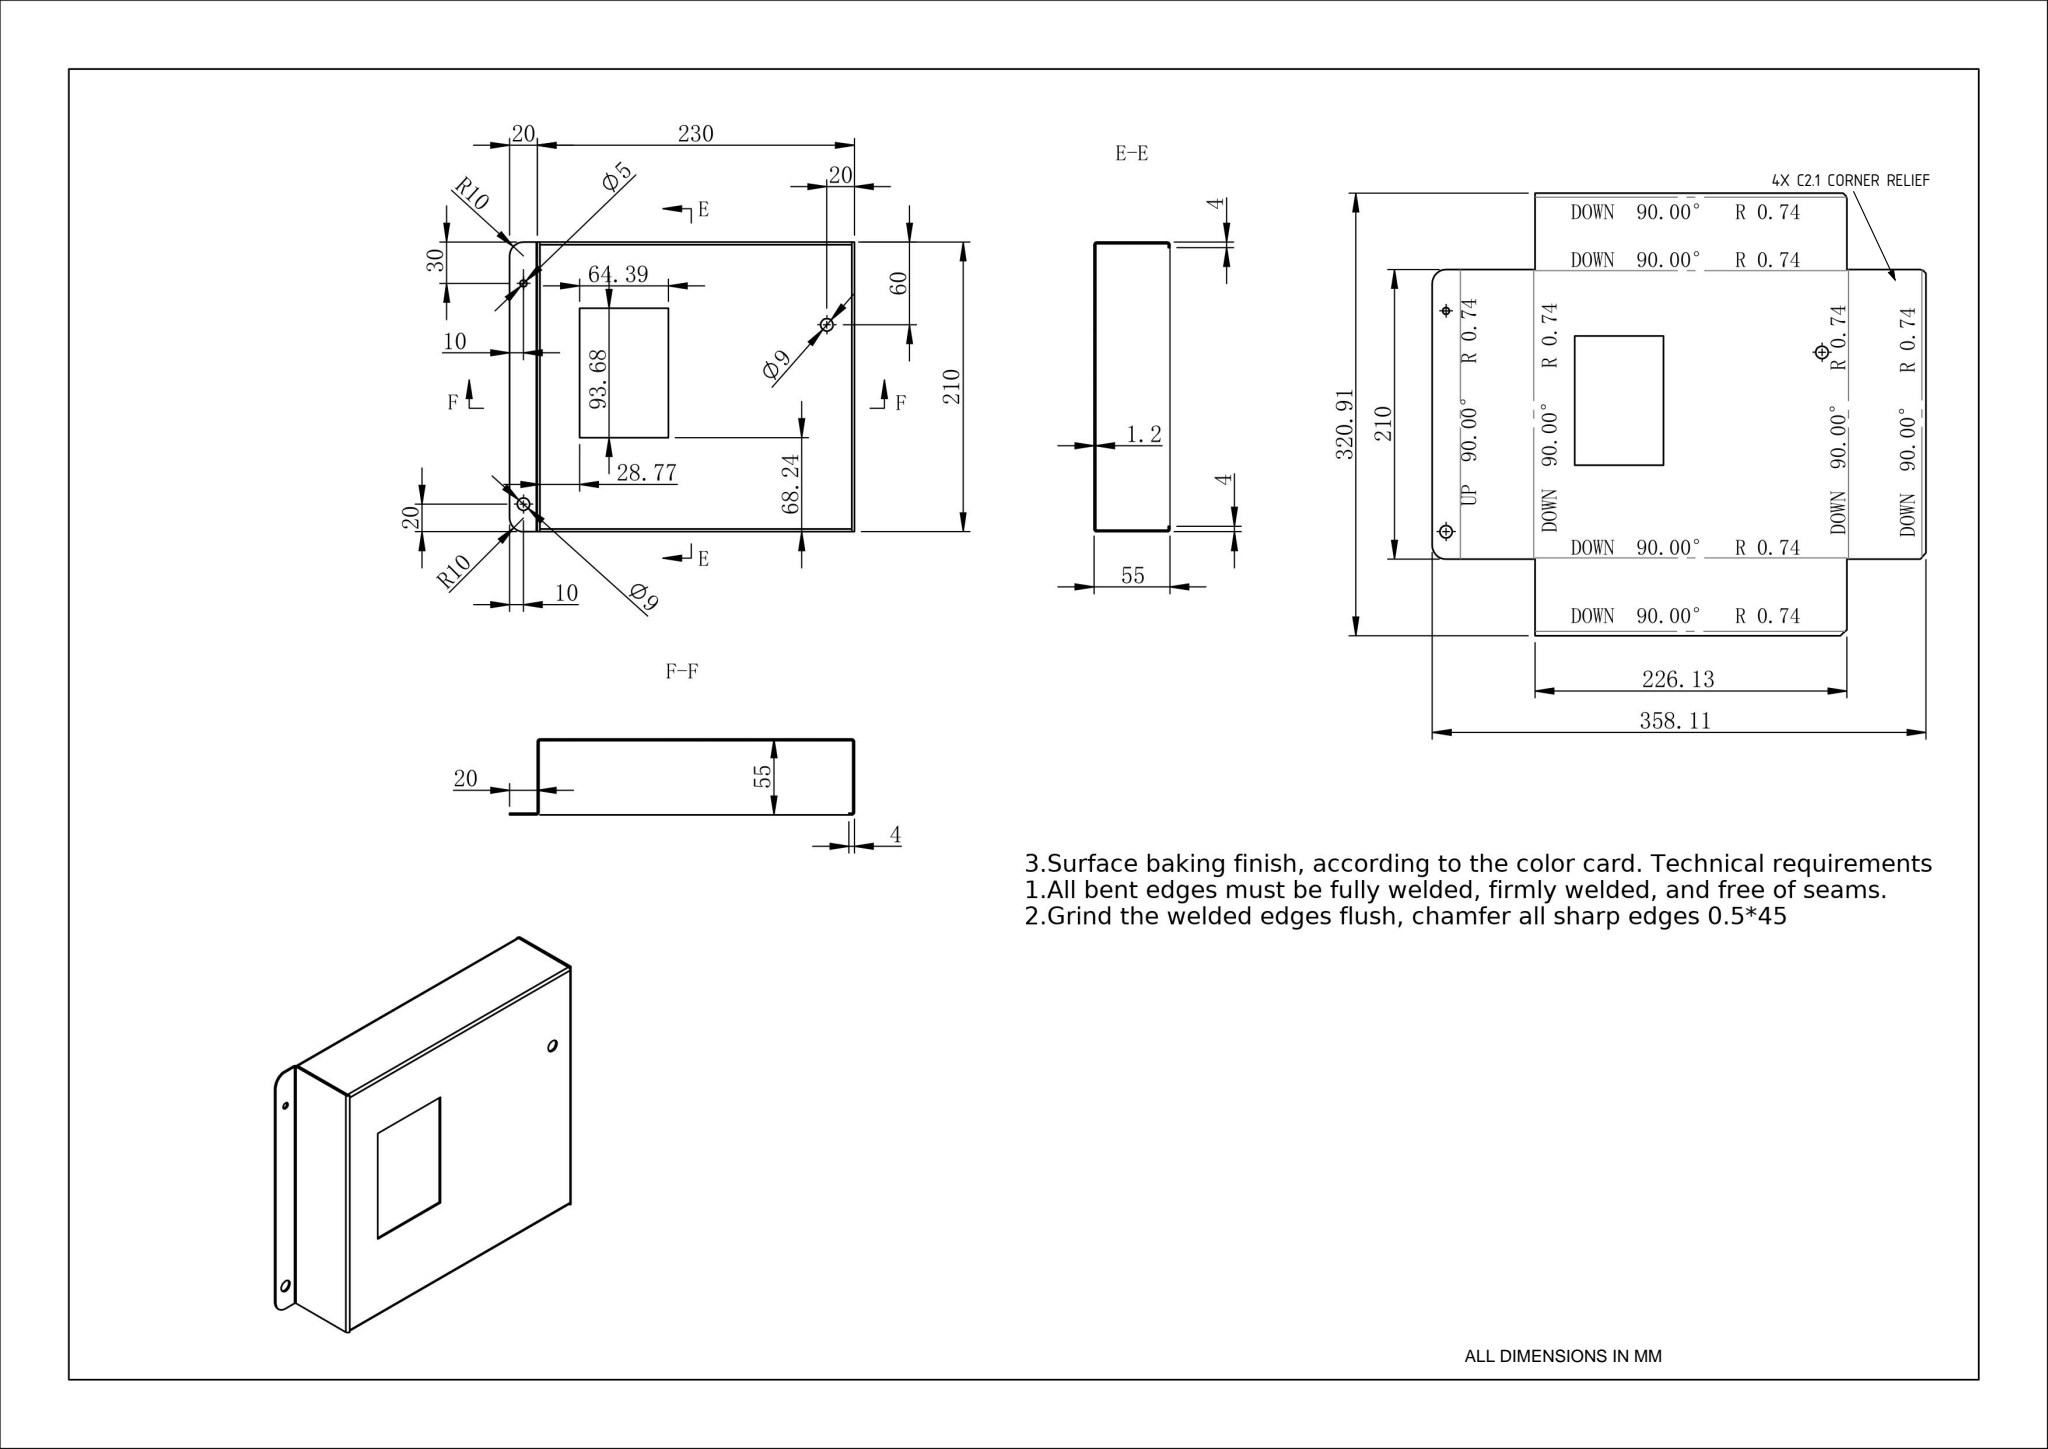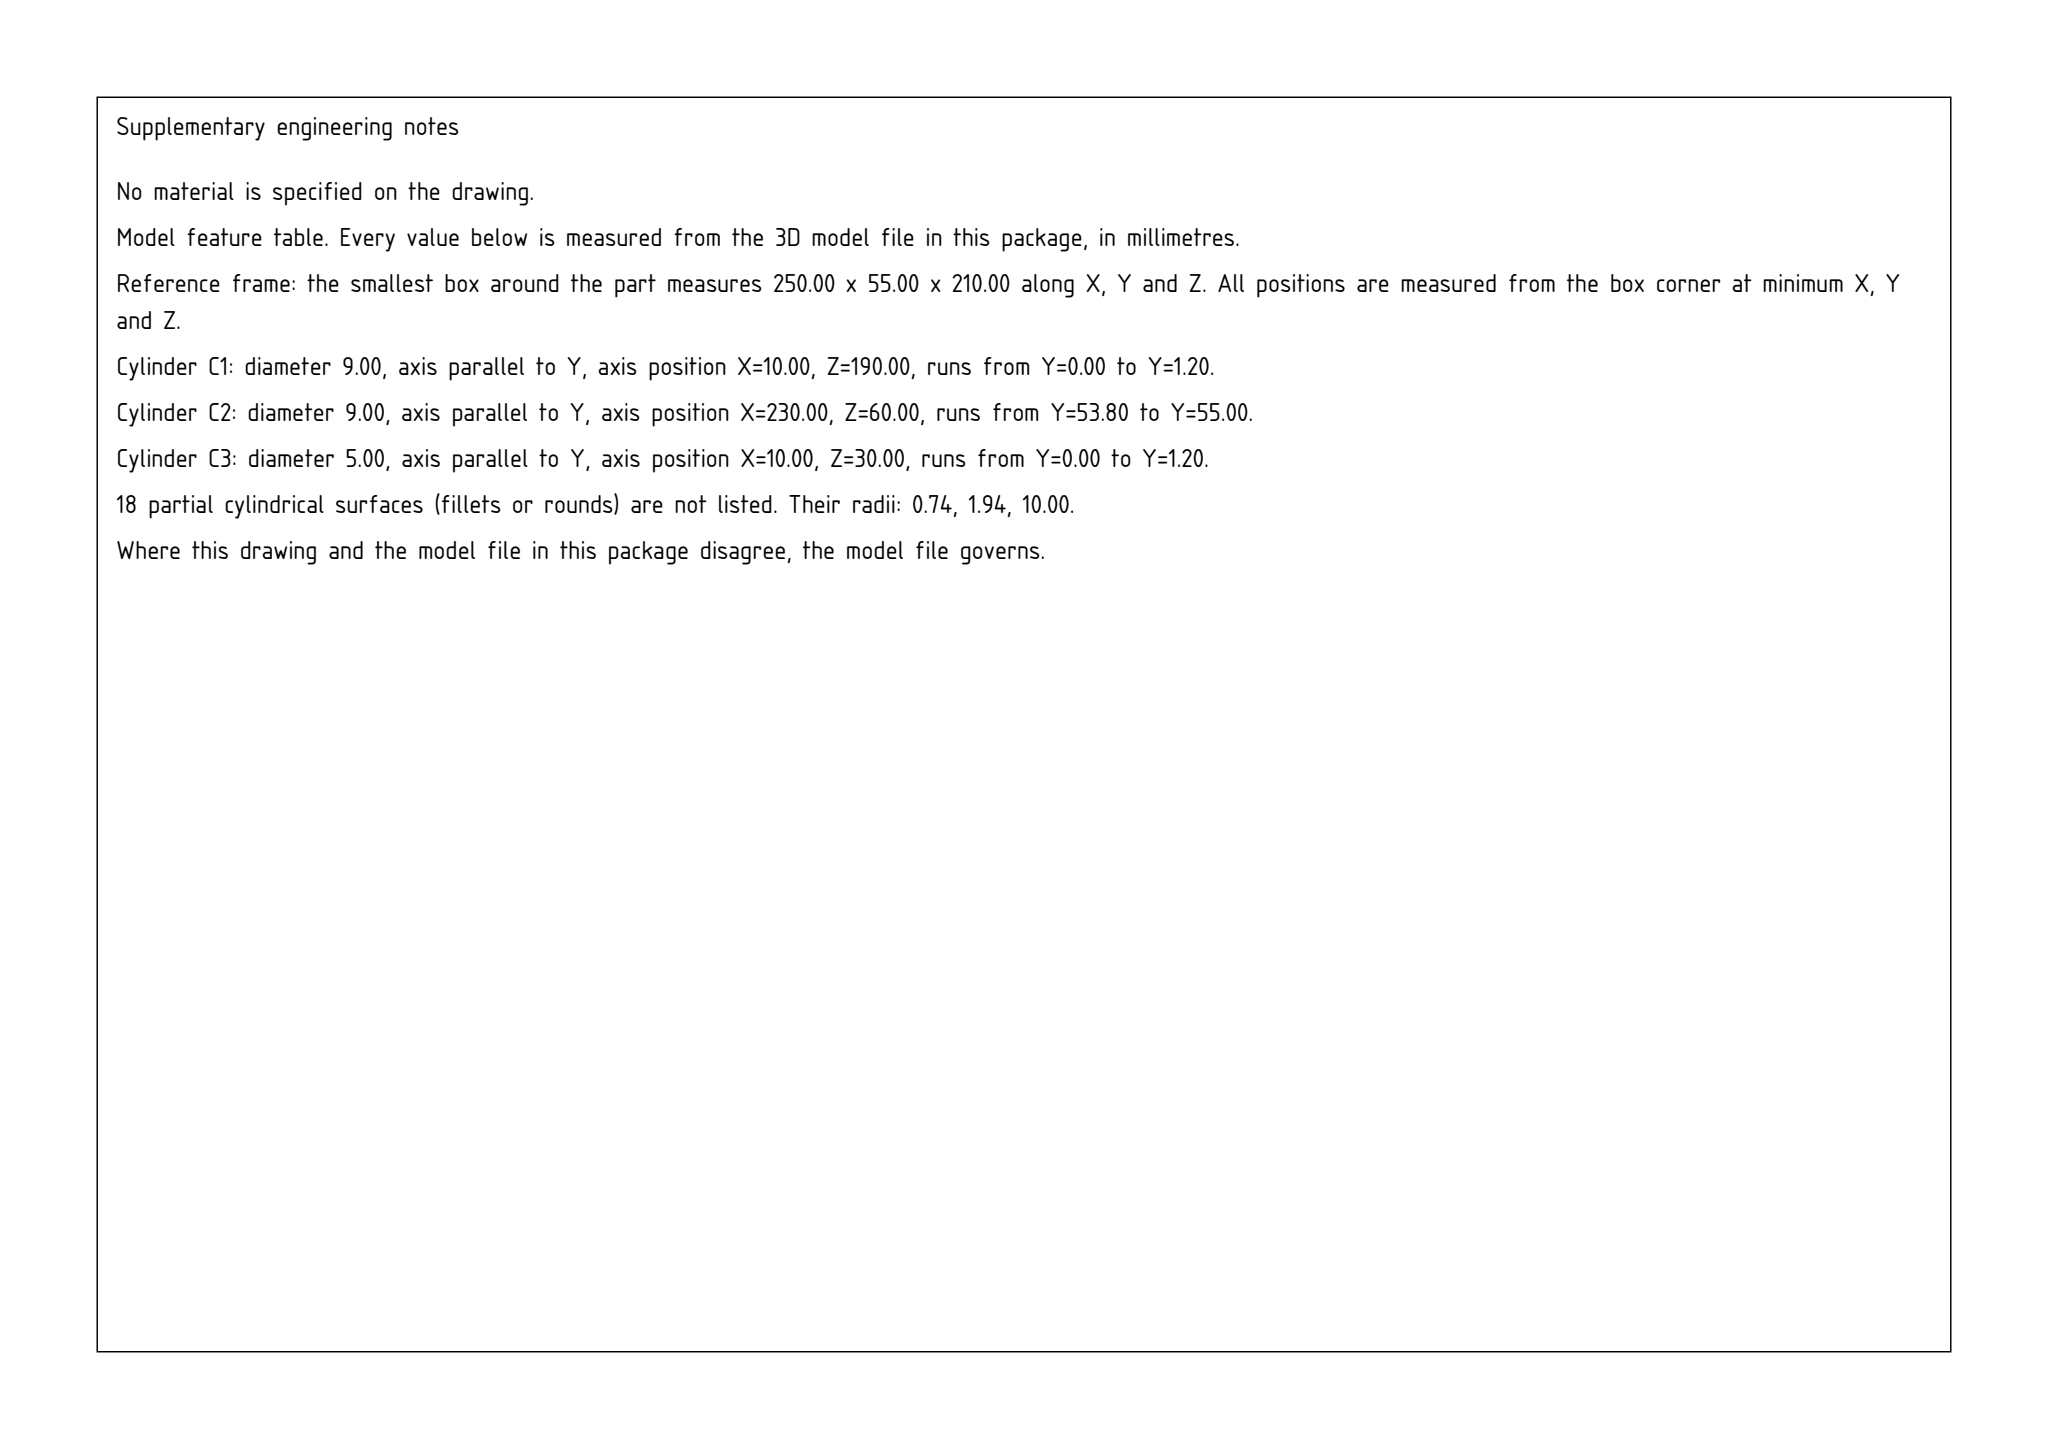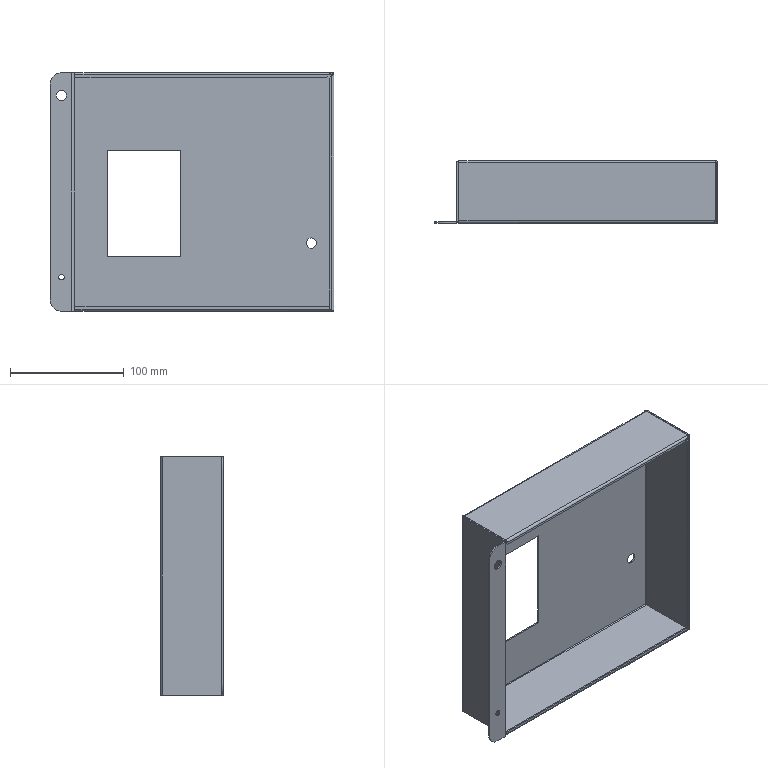Part | SolidWorks | mm | 1 solid | 86 faces | box 250 x 55 x 210 mm | volume 112835 mm3 | plane 58 | cylinder 24 | spline 4 | commonest cylinder face diameters 3.873 x8 1.473 x8 9 x4 5 x2 20 x2
Drawing notes:
FLAT PATTERN: 4X C2.1 (45°) CORNER RELIEF AT RH LIP/TOP & BTM LIPS | from the solid: 4 inclined planes at 45°/90°/45°, size 2.1 x 1.2 x 2.1, at bbox_from [243.4,0,206.0], [245.3,0,1.9], [246.0,0,0.7], [246.0,0,205.3] - corners of x=246.0 RH lip face (y 0-1.2) meeting z=4.0 and z=206.0 lip faces